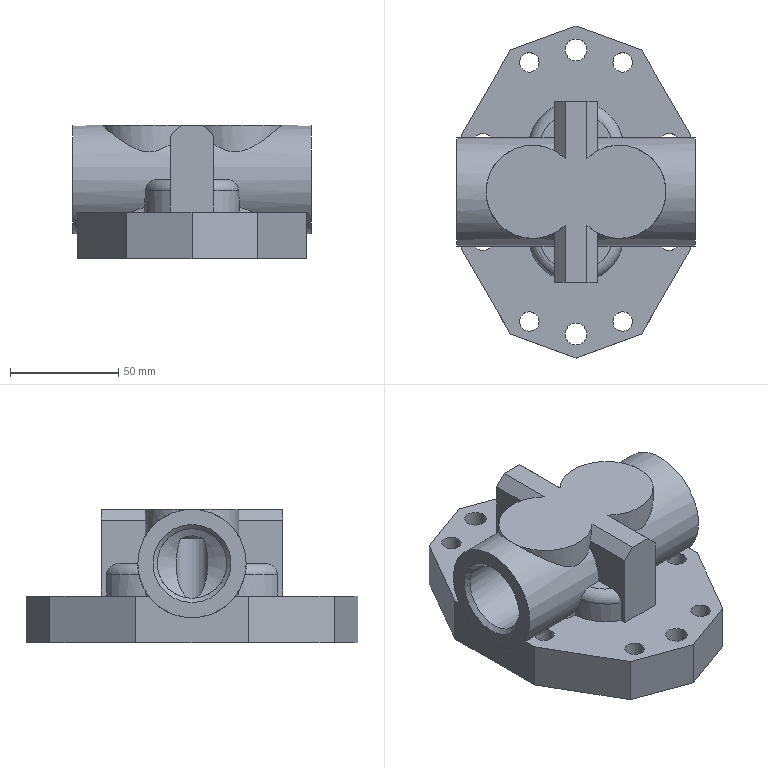Component | NX | CYCH_1_REARPUMPCOVER | 1 solid | 77 faces | volume 395193 mm3 | plane 32 | cylinder 30 | cone 9 | torus 4 | other 2 | commonest cylinder face diameters 43 x8 9 x8 44 x4 10 x2 50 x2 25 x2 19 x1 15 x1